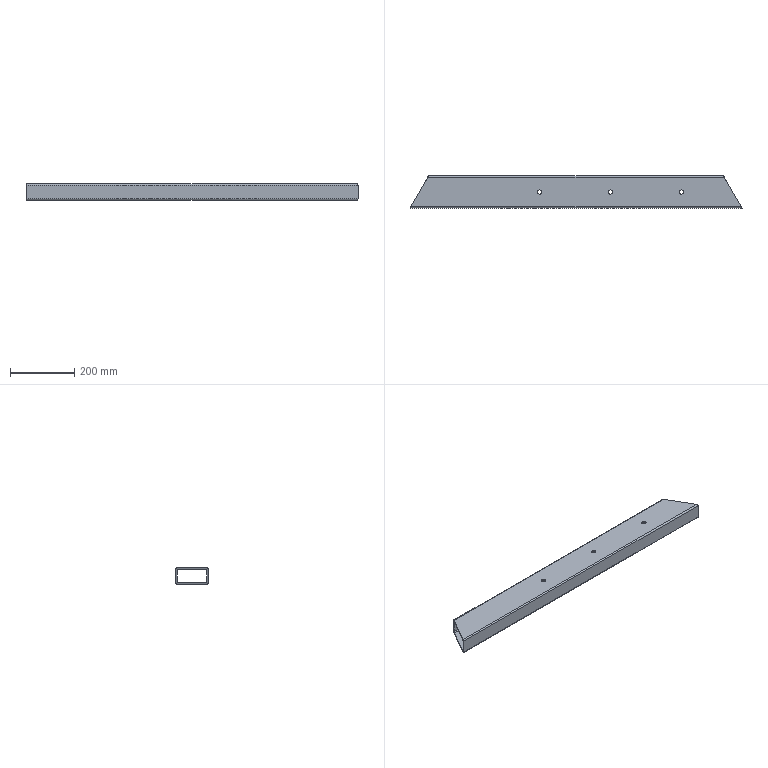Component | NX | INCL_SUPP_FRAME_BOT_BEAM | 1 solid | 24 faces | volume 1101307 mm3 | cylinder 14 | plane 10 | commonest cylinder face diameters 8 x8 13 x6